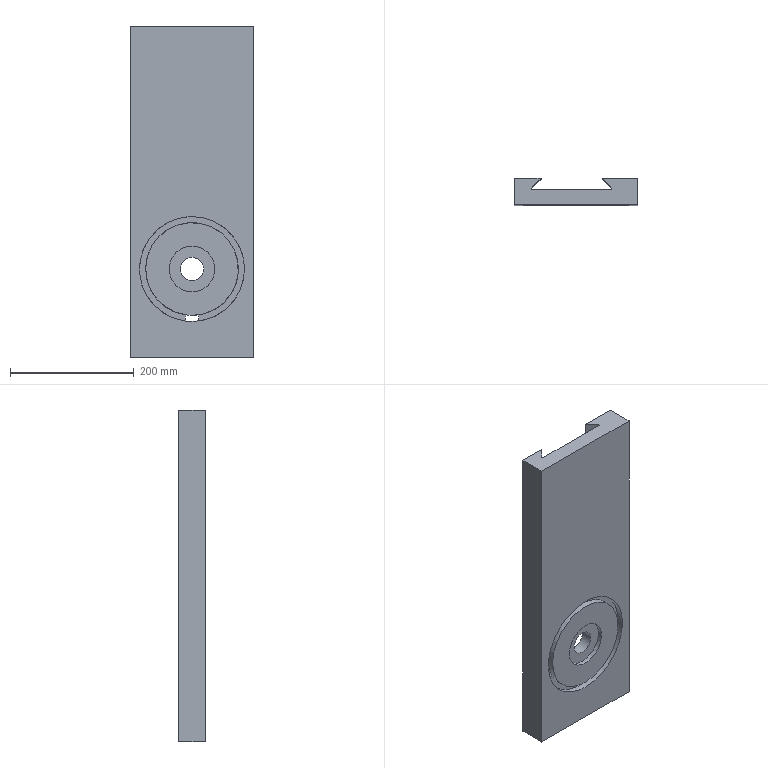Component | NX | DOVETAIL_SEAT | 1 solid | 24 faces | volume 3407526 mm3 | plane 18 | cylinder 6 | commonest cylinder face diameters 22 x2 170 x1 150 x1 74 x1 38 x1